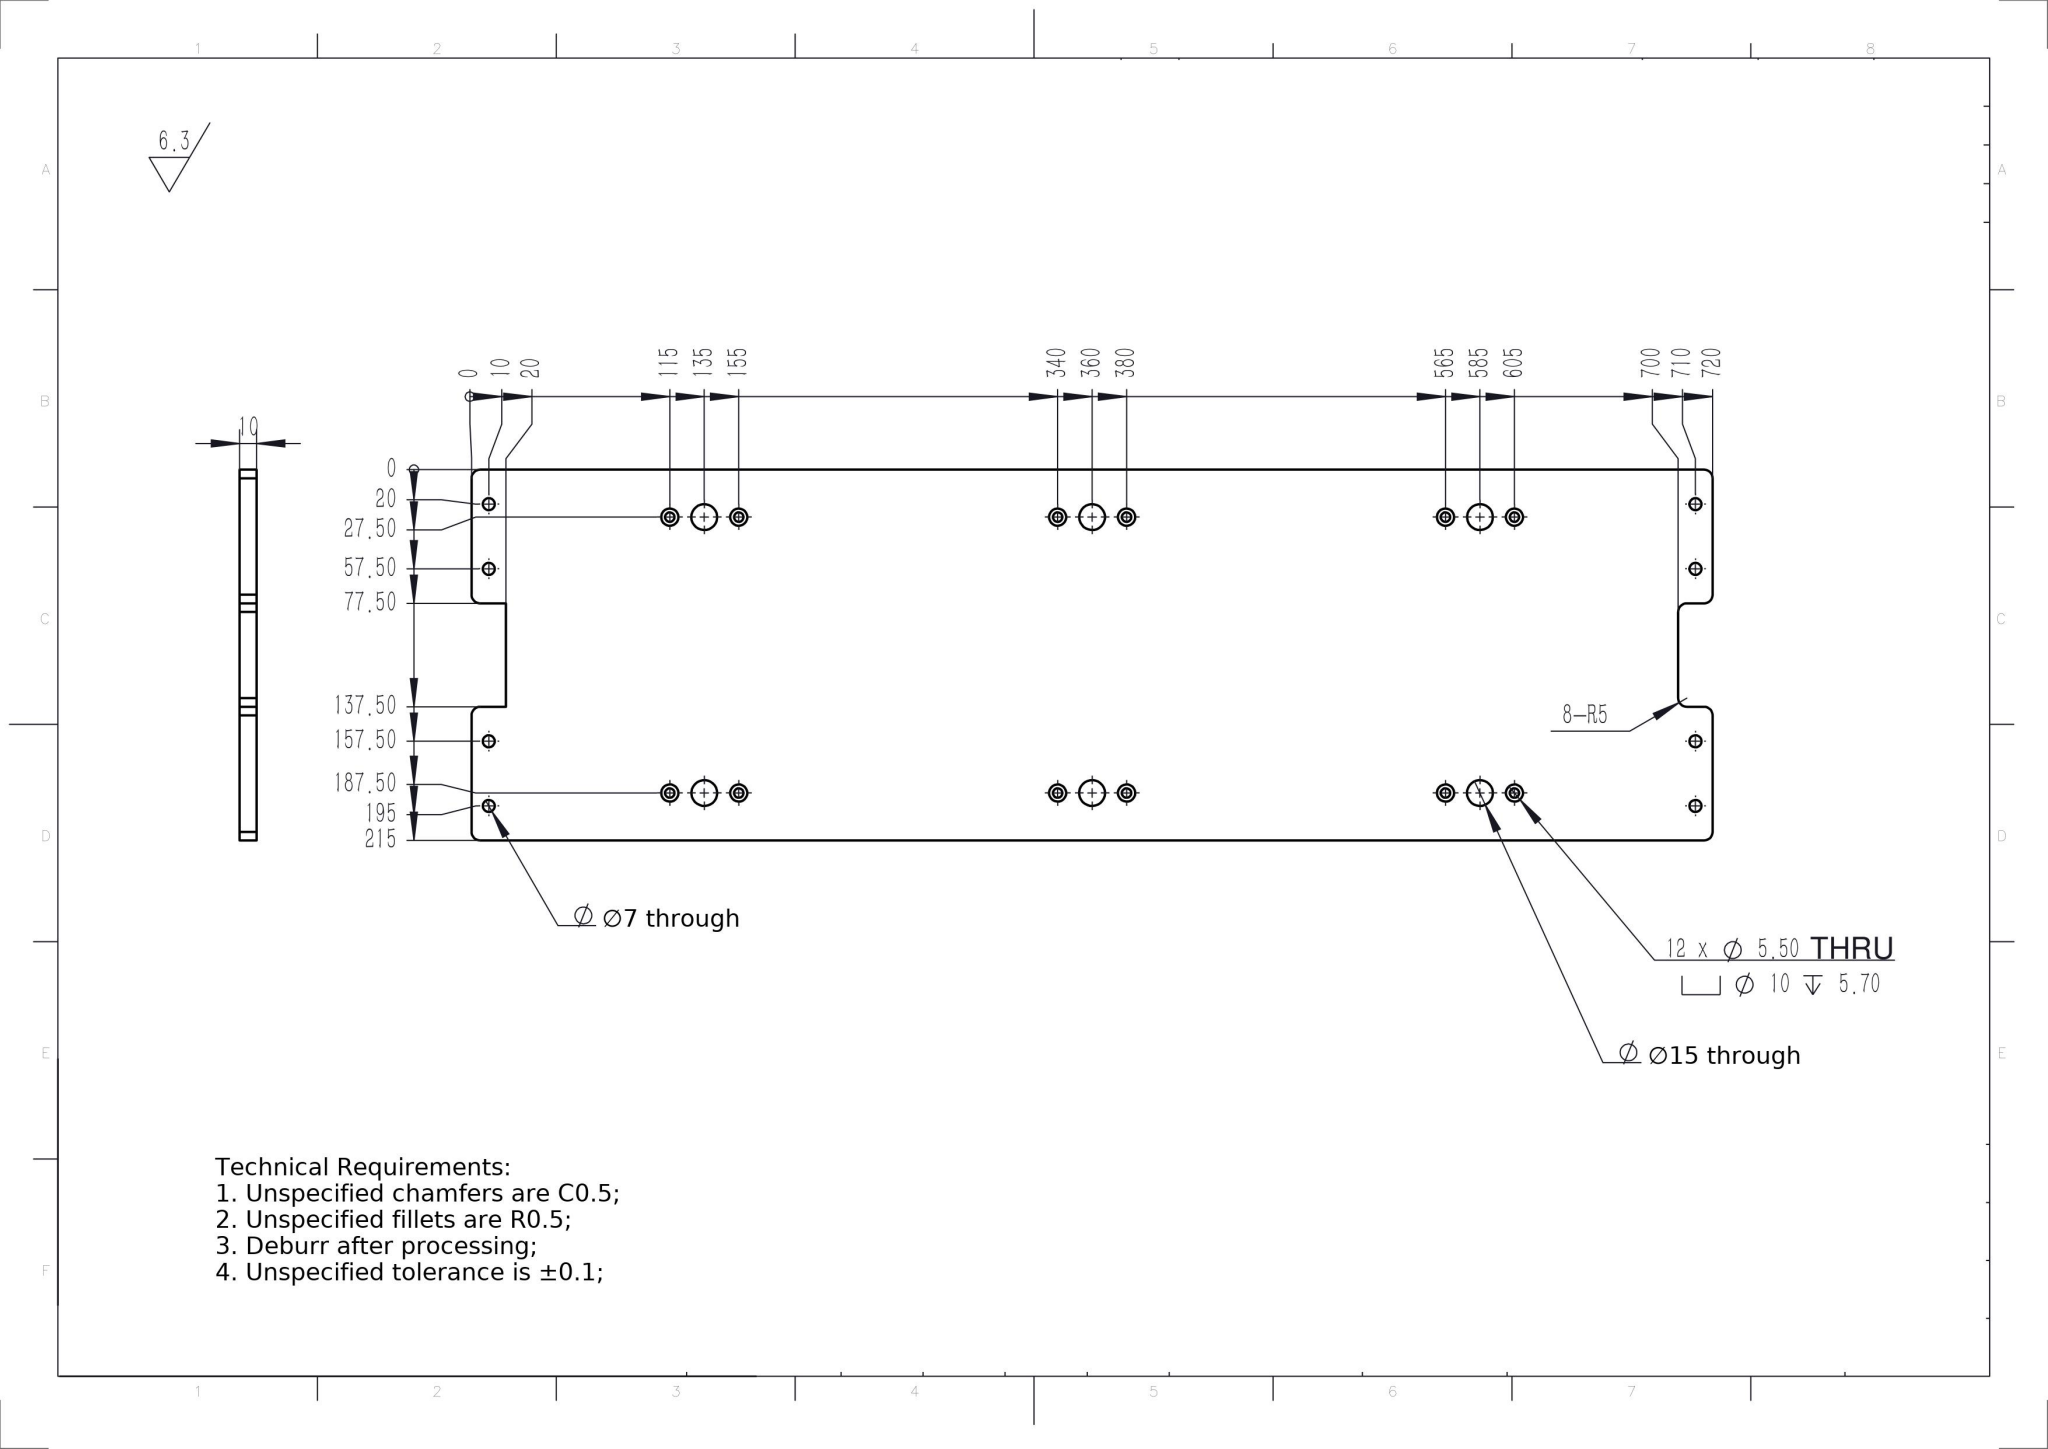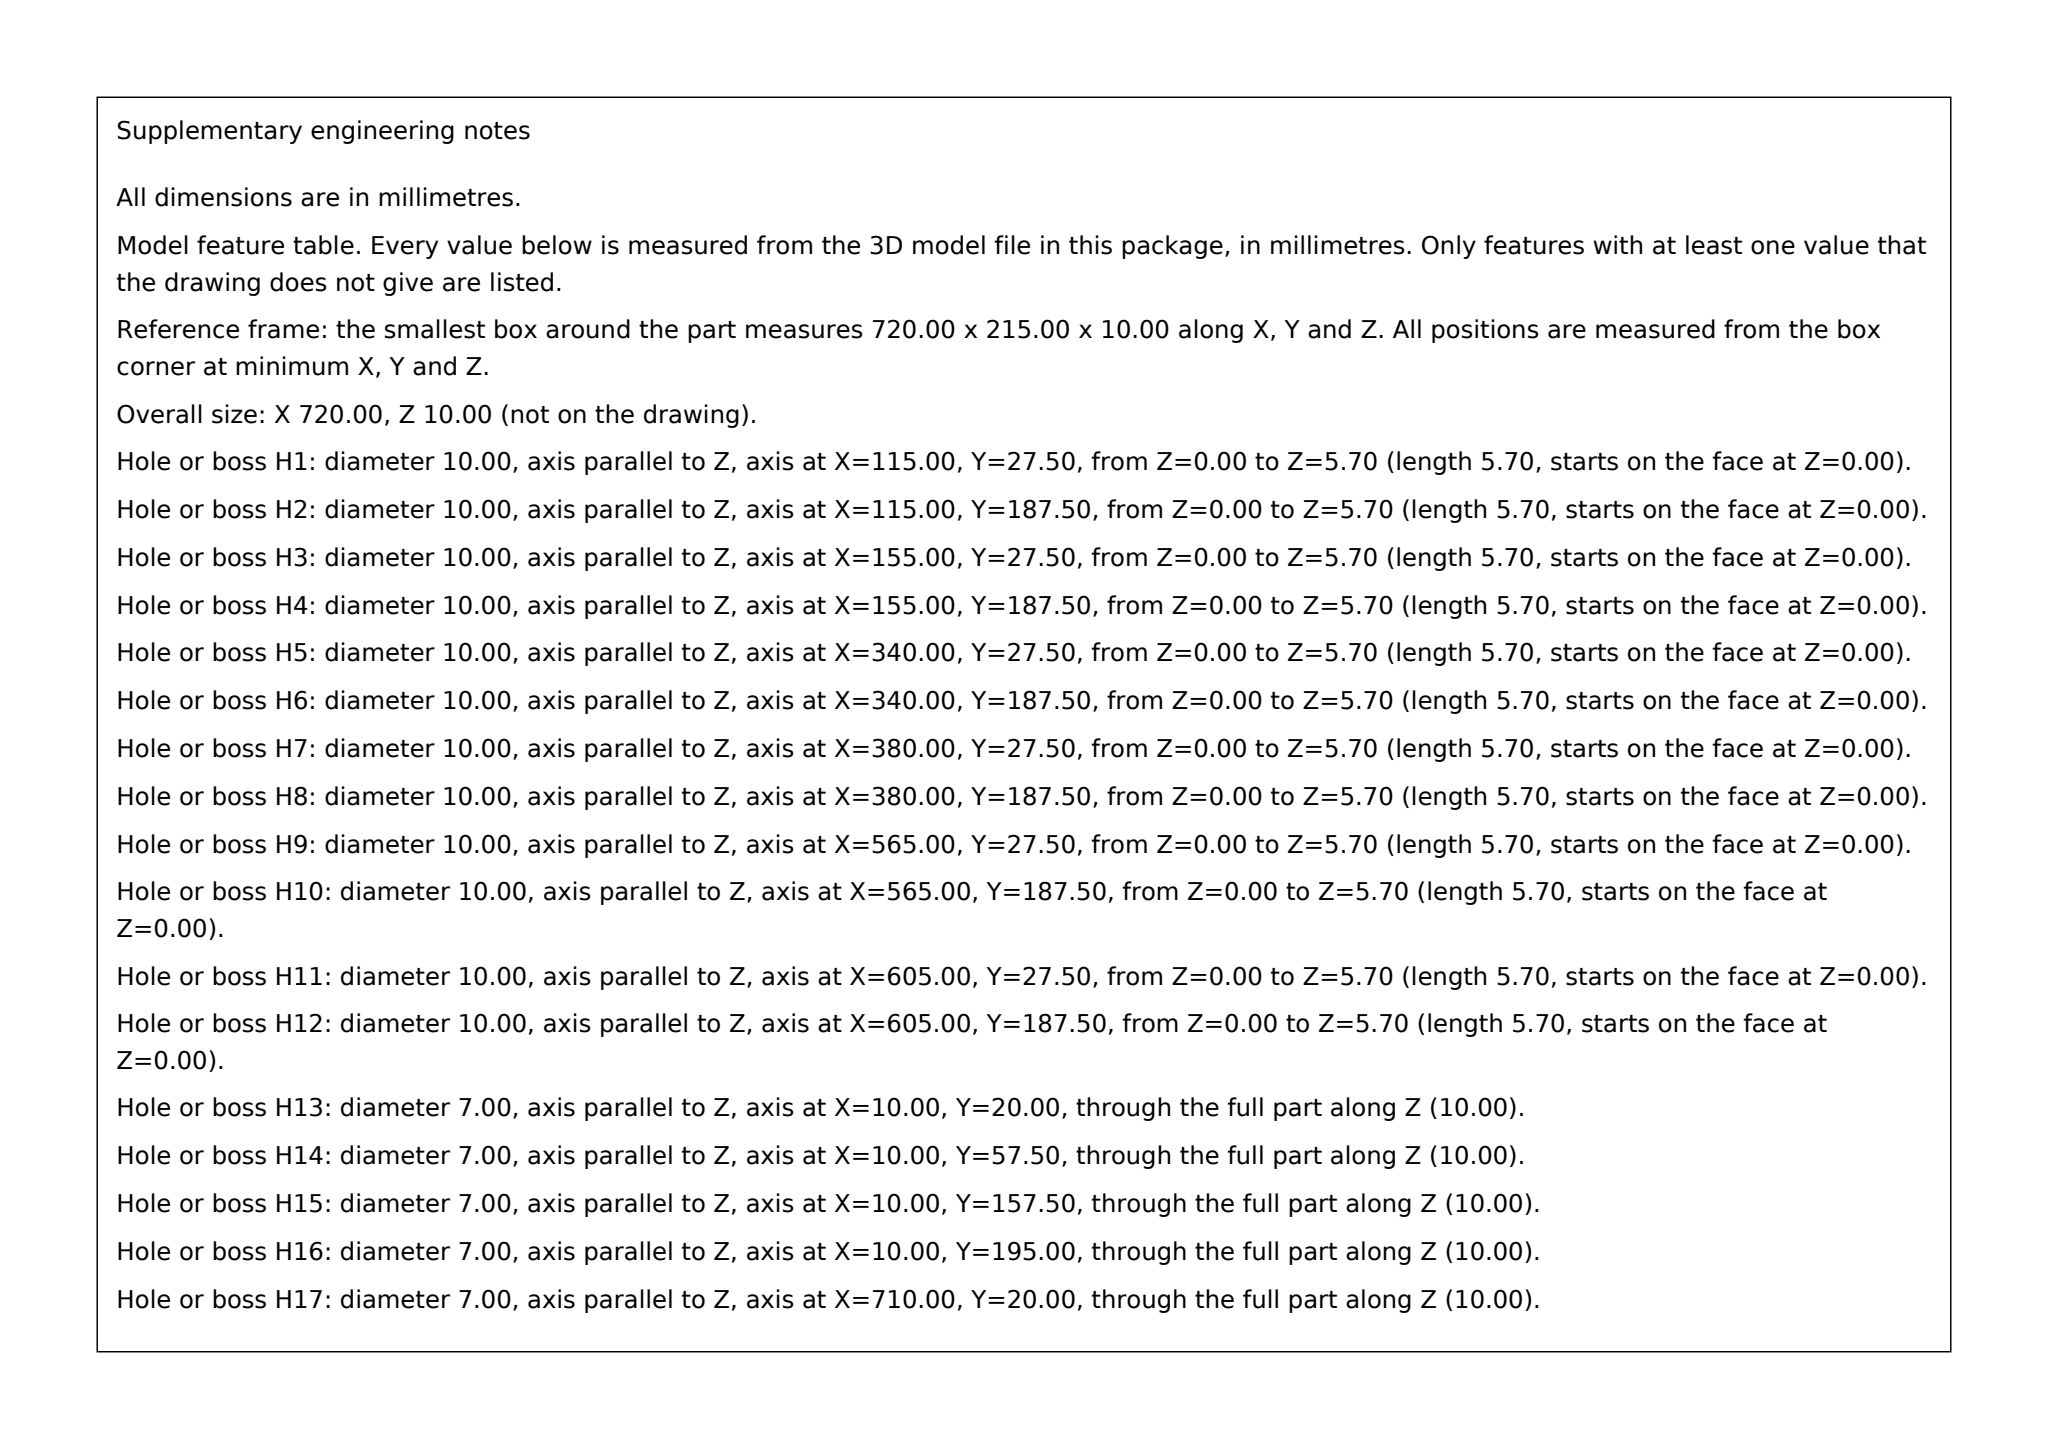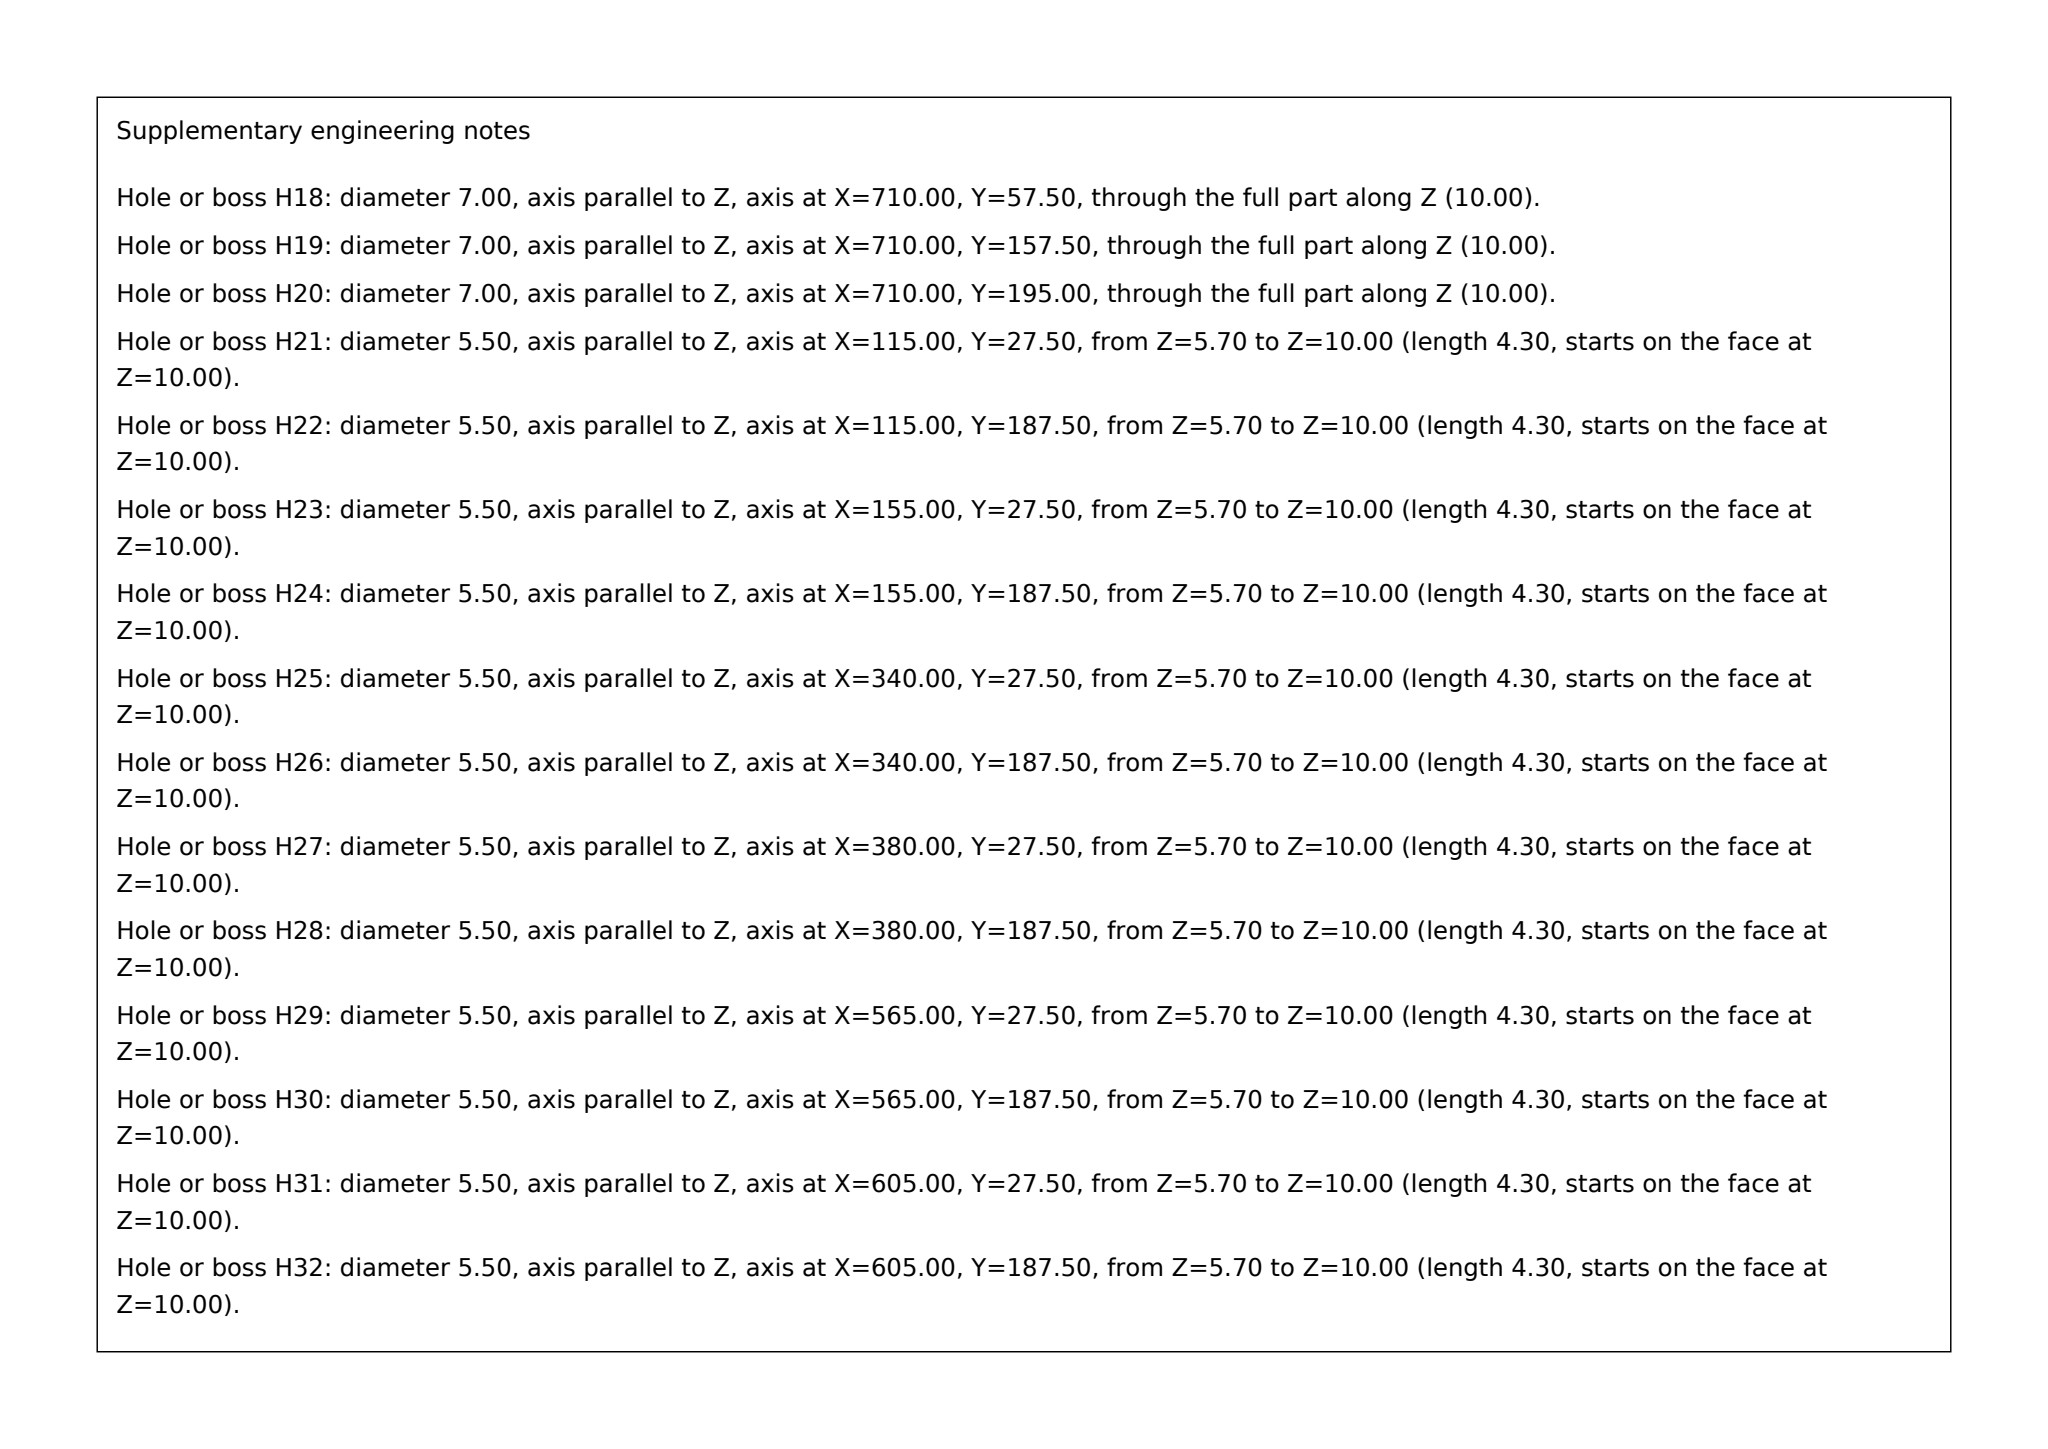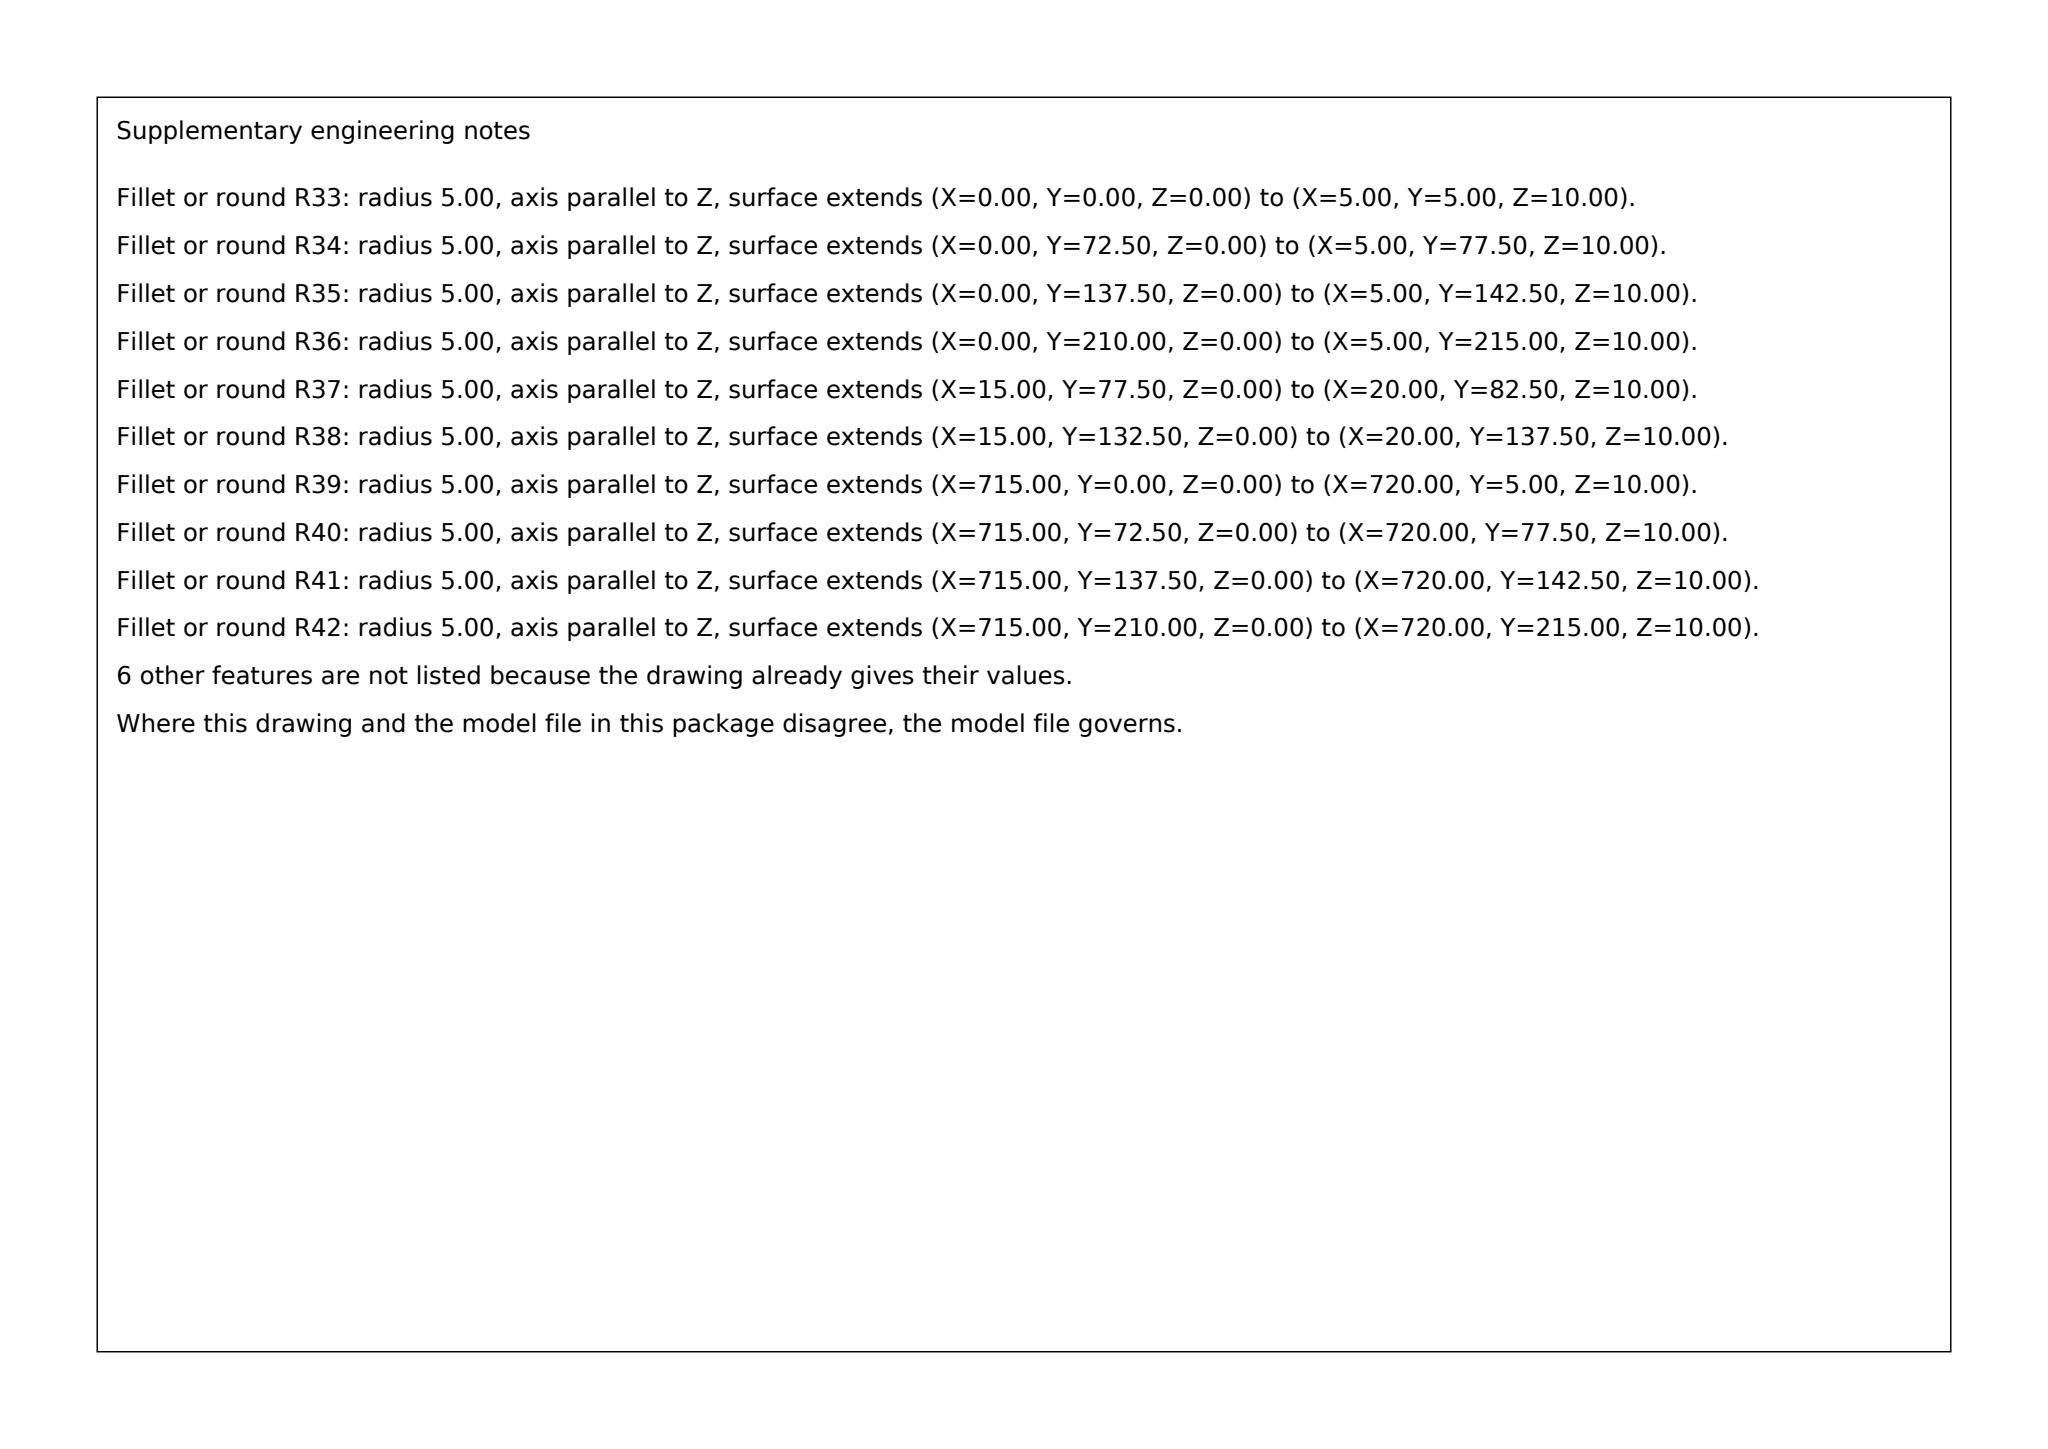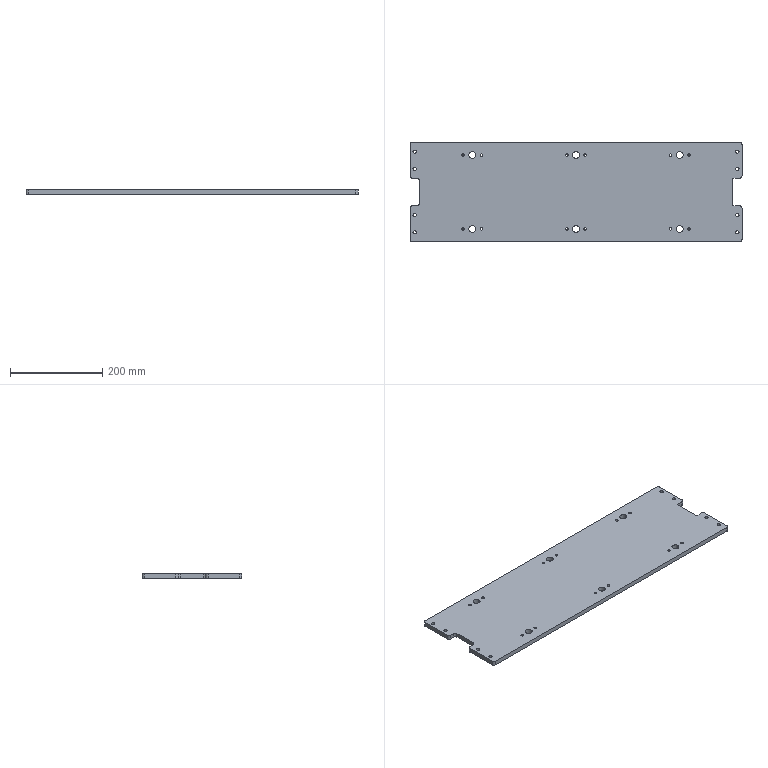Part | SolidWorks | mm | 1 solid | 112 faces | box 720 x 215 x 10 mm | volume 1503398 mm3 | cylinder 86 | plane 26 | commonest cylinder face diameters 10 x34 5.5 x24 7 x16 15 x12
build123d program:
from build123d import *

# Parameters (mm, degrees)
SKETCH1_W                                         = 720
SKETCH1_H                                         = 215
BOSS_EXTRUDE1_DEPTH                               = 10
SKETCH2_W                                         = 20
SKETCH2_H                                         = 60
CUT_EXTRUDE1_DEPTH                                = 10
FILLET1_R                                         = 5
SKETCH3_R                                         = 3.5
CUT_EXTRUDE2_DEPTH                                = 10
FILLET2_R                                         = 5
SKETCH4_R                                         = 7.5
CUT_EXTRUDE3_DEPTH                                = 10
HOLE_SIZE_ACCORDING_TO_HEXAGON_SOCKET_D           = 5.5
HOLE_SIZE_ACCORDING_TO_HEXAGON_SOCKET_CBORE_D     = 10
HOLE_SIZE_ACCORDING_TO_HEXAGON_SOCKET_CBORE_DEPTH = 5.7


with BuildPart() as part:
    # Sketch1 → Boss-Extrude1 (new body)
    with BuildSketch(Plane.XY):
        Rectangle(SKETCH1_W, SKETCH1_H)
    extrude(amount=BOSS_EXTRUDE1_DEPTH)

    # Sketch2 → Cut-Extrude1 (cut)
    with BuildSketch(Plane.XY.offset(10)):
        with Locations((-350, 0)):
            Rectangle(SKETCH2_W, SKETCH2_H)
        with Locations((350, 0)):
            Rectangle(SKETCH2_W, SKETCH2_H)
    extrude(amount=-CUT_EXTRUDE1_DEPTH, mode=Mode.SUBTRACT)

    # Fillet1
    fillet1_edges = [part.edges().sort_by_distance(p)[0] for p in [
        (-340, 30, 5),
        (-340, -30, 5),
    ]]
    fillet(fillet1_edges, radius=FILLET1_R)

    # Sketch3 → Cut-Extrude2 (cut)
    with BuildSketch(Plane.XY.offset(10)):
        with Locations((-350, 87.5)):
            Circle(SKETCH3_R)
        with Locations((-350, 50)):
            Circle(SKETCH3_R)
        with Locations(Location((-350, -50, 0), (0, 0, 180))):
            Circle(SKETCH3_R)
        with Locations(Location((-350, -87.5, 0), (0, 0, 180))):
            Circle(SKETCH3_R)
        with Locations((350, -87.5)):
            Circle(SKETCH3_R)
        with Locations((350, -50)):
            Circle(SKETCH3_R)
        with Locations(Location((350, 50, 0), (0, 0, 180))):
            Circle(SKETCH3_R)
        with Locations(Location((350, 87.5, 0), (0, 0, 180))):
            Circle(SKETCH3_R)
    extrude(amount=-CUT_EXTRUDE2_DEPTH, mode=Mode.SUBTRACT)

    # Fillet2
    fillet2_edges = [part.edges().sort_by_distance(p)[0] for p in [
        (-360, -30, 5),
        (-360, 30, 5),
        (360, 30, 5),
        (360, -30, 5),
        (360, -107.5, 5),
        (-360, -107.5, 5),
        (-360, 107.5, 5),
        (360, 107.5, 5),
    ]]
    fillet(fillet2_edges, radius=FILLET2_R)

    # Sketch4 → Cut-Extrude3 (cut)
    with BuildSketch(Plane.XY.offset(10)):
        with Locations((225, 80)):
            Circle(SKETCH4_R)
        with Locations((0, 80)):
            Circle(SKETCH4_R)
        with Locations(Location((-225, 80, 0), (0, 0, 180))):
            Circle(SKETCH4_R)
        with Locations((-225, -80)):
            Circle(SKETCH4_R)
        with Locations(Location((0, -80, 0), (0, 0, 180))):
            Circle(SKETCH4_R)
        with Locations(Location((225, -80, 0), (0, 0, 180))):
            Circle(SKETCH4_R)
    extrude(amount=-CUT_EXTRUDE3_DEPTH, mode=Mode.SUBTRACT)

    # Hole Size _ according to_ Hexagon Socket (through all)
    with Locations(Plane(origin=(0, 0, 0), x_dir=(1, 0, 0), z_dir=(0, 0, -1))):
        with Locations((245, 80), (205, 80), (20, 80), (-20, 80), (-205, 80), (-245, 80), (20, -80), (-20, -80), (-205, -80), (-245, -80), (245, -80), (205, -80)):
            CounterBoreHole(HOLE_SIZE_ACCORDING_TO_HEXAGON_SOCKET_D / 2, HOLE_SIZE_ACCORDING_TO_HEXAGON_SOCKET_CBORE_D / 2, HOLE_SIZE_ACCORDING_TO_HEXAGON_SOCKET_CBORE_DEPTH)


solid = part.part